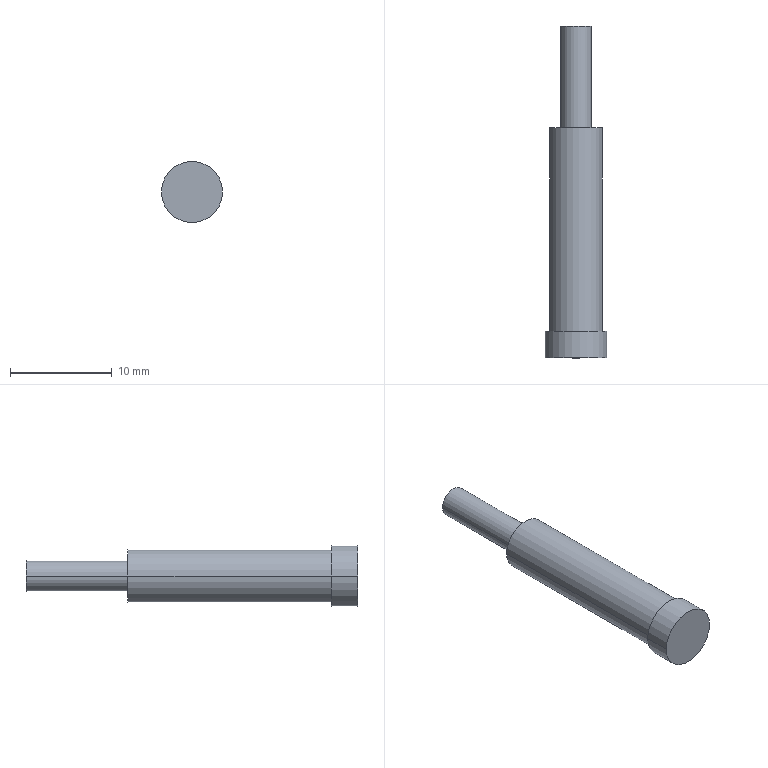Component | SolidWorks | FQ-10-1 | 1 solid | 10 faces | box 6 x 32.6 x 6 mm | volume 569 mm3 | cylinder 6 | plane 4 | commonest cylinder face diameters 3 x2 5.2 x2 6 x2
build123d program:
from build123d import *

# Parameters (mm, degrees)
SKETCH1_R           = 3
BOSS_EXTRUDE1_DEPTH = 2.6
SKETCH2_R           = 2.6
BOSS_EXTRUDE2_DEPTH = 20
SKETCH3_R           = 1.5
BOSS_EXTRUDE3_DEPTH = 10


with BuildPart() as part:
    # Sketch1 → Boss-Extrude1 (new body)
    with BuildSketch(Plane.XY):
        Circle(SKETCH1_R)
    extrude(amount=BOSS_EXTRUDE1_DEPTH)

    # Sketch2 → Boss-Extrude2 (add)
    with BuildSketch(Plane.XY.offset(2.6)):
        Circle(SKETCH2_R)
    extrude(amount=BOSS_EXTRUDE2_DEPTH)

    # Sketch3 → Boss-Extrude3 (add)
    with BuildSketch(Plane.XY.offset(22.6)):
        Circle(SKETCH3_R)
    extrude(amount=BOSS_EXTRUDE3_DEPTH)


solid = part.part

# Placed as in the assembly
solid = solid.moved(Location((-102.663, 0.3959, 98.5), (-90, 0, 0)))
STEP:
#1=COLOUR_RGB('',0.7922,0.8196,0.9333);
#2=FILL_AREA_STYLE_COLOUR('',#1);
#3=FILL_AREA_STYLE('',(#2));
#4=SURFACE_STYLE_FILL_AREA(#3);
#5=SURFACE_SIDE_STYLE('',(#4));
#6=SURFACE_STYLE_USAGE(.BOTH.,#5);
#7=PRESENTATION_STYLE_ASSIGNMENT((#6));
#8=CARTESIAN_POINT('',(-3.983,1.299,3.878));
#9=VERTEX_POINT('',#8);
#10=CARTESIAN_POINT('',(-4.101,1.299,3.878));
#11=VERTEX_POINT('',#10);
#12=CARTESIAN_POINT('',(-4.042,1.299,3.878));
#13=DIRECTION('',(0.,1.,0.));
#14=DIRECTION('',(1.,0.,0.));
#15=AXIS2_PLACEMENT_3D('',#12,#13,#14);
#16=CIRCLE('',#15,0.05906);
#17=EDGE_CURVE('',#9,#11,#16,.T.);
#18=ORIENTED_EDGE('',*,*,#17,.F.);
#19=CARTESIAN_POINT('',(-3.983,0.9054,3.878));
#20=VERTEX_POINT('',#19);
#21=CARTESIAN_POINT('',(-3.983,1.299,3.878));
#22=DIRECTION('',(0.,-1.,0.));
#23=VECTOR('',#22,39.37);
#24=LINE('',#21,#23);
#25=EDGE_CURVE('',#9,#20,#24,.T.);
#26=ORIENTED_EDGE('',*,*,#25,.T.);
#27=CARTESIAN_POINT('',(-4.101,0.9054,3.878));
#28=VERTEX_POINT('',#27);
#29=CARTESIAN_POINT('',(-4.042,0.9054,3.878));
#30=DIRECTION('',(0.,1.,0.));
#31=DIRECTION('',(1.,0.,0.));
#32=AXIS2_PLACEMENT_3D('',#29,#30,#31);
#33=CIRCLE('',#32,0.05906);
#34=EDGE_CURVE('',#20,#28,#33,.T.);
#35=ORIENTED_EDGE('',*,*,#34,.T.);
#36=CARTESIAN_POINT('',(-4.101,1.299,3.878));
#37=DIRECTION('',(0.,-1.,0.));
#38=VECTOR('',#37,39.37);
#39=LINE('',#36,#38);
#40=EDGE_CURVE('',#11,#28,#39,.T.);
#41=ORIENTED_EDGE('',*,*,#40,.F.);
#42=EDGE_LOOP('',(#18,#26,#35,#41));
#43=FACE_OUTER_BOUND('',#42,.T.);
#44=CARTESIAN_POINT('',(-4.042,1.299,3.878));
#45=DIRECTION('',(0.,-1.,0.));
#46=DIRECTION('',(-1.,0.,0.));
#47=AXIS2_PLACEMENT_3D('',#44,#45,#46);
#48=CYLINDRICAL_SURFACE('',#47,0.05906);
#49=ADVANCED_FACE('',(#43),#48,.T.);
#50=CARTESIAN_POINT('',(-3.94,0.9054,3.878));
#51=VERTEX_POINT('',#50);
#52=CARTESIAN_POINT('',(-4.144,0.9054,3.878));
#53=VERTEX_POINT('',#52);
#54=CARTESIAN_POINT('',(-4.042,0.9054,3.878));
#55=DIRECTION('',(0.,1.,0.));
#56=DIRECTION('',(1.,0.,0.));
#57=AXIS2_PLACEMENT_3D('',#54,#55,#56);
#58=CIRCLE('',#57,0.1024);
#59=EDGE_CURVE('',#51,#53,#58,.T.);
#60=ORIENTED_EDGE('',*,*,#59,.F.);
#61=CARTESIAN_POINT('',(-3.94,0.118,3.878));
#62=VERTEX_POINT('',#61);
#63=CARTESIAN_POINT('',(-3.94,0.9054,3.878));
#64=DIRECTION('',(0.,-1.,0.));
#65=VECTOR('',#64,39.37);
#66=LINE('',#63,#65);
#67=EDGE_CURVE('',#51,#62,#66,.T.);
#68=ORIENTED_EDGE('',*,*,#67,.T.);
#69=CARTESIAN_POINT('',(-4.144,0.118,3.878));
#70=VERTEX_POINT('',#69);
#71=CARTESIAN_POINT('',(-4.042,0.118,3.878));
#72=DIRECTION('',(0.,1.,0.));
#73=DIRECTION('',(1.,0.,0.));
#74=AXIS2_PLACEMENT_3D('',#71,#72,#73);
#75=CIRCLE('',#74,0.1024);
#76=EDGE_CURVE('',#62,#70,#75,.T.);
#77=ORIENTED_EDGE('',*,*,#76,.T.);
#78=CARTESIAN_POINT('',(-4.144,0.9054,3.878));
#79=DIRECTION('',(0.,-1.,0.));
#80=VECTOR('',#79,39.37);
#81=LINE('',#78,#80);
#82=EDGE_CURVE('',#53,#70,#81,.T.);
#83=ORIENTED_EDGE('',*,*,#82,.F.);
#84=EDGE_LOOP('',(#60,#68,#77,#83));
#85=FACE_OUTER_BOUND('',#84,.T.);
#86=CARTESIAN_POINT('',(-4.042,0.9054,3.878));
#87=DIRECTION('',(0.,-1.,0.));
#88=DIRECTION('',(-1.,0.,0.));
#89=AXIS2_PLACEMENT_3D('',#86,#87,#88);
#90=CYLINDRICAL_SURFACE('',#89,0.1024);
#91=ADVANCED_FACE('',(#85),#90,.T.);
#92=CARTESIAN_POINT('',(-3.924,0.118,3.878));
#93=VERTEX_POINT('',#92);
#94=CARTESIAN_POINT('',(-4.16,0.118,3.878));
#95=VERTEX_POINT('',#94);
#96=CARTESIAN_POINT('',(-4.042,0.118,3.878));
#97=DIRECTION('',(0.,1.,0.));
#98=DIRECTION('',(1.,0.,0.));
#99=AXIS2_PLACEMENT_3D('',#96,#97,#98);
#100=CIRCLE('',#99,0.1181);
#101=EDGE_CURVE('',#93,#95,#100,.T.);
#102=ORIENTED_EDGE('',*,*,#101,.F.);
#103=CARTESIAN_POINT('',(-3.924,0.01559,3.878));
#104=VERTEX_POINT('',#103);
#105=CARTESIAN_POINT('',(-3.924,0.118,3.878));
#106=DIRECTION('',(0.,-1.,0.));
#107=VECTOR('',#106,39.37);
#108=LINE('',#105,#107);
#109=EDGE_CURVE('',#93,#104,#108,.T.);
#110=ORIENTED_EDGE('',*,*,#109,.T.);
#111=CARTESIAN_POINT('',(-4.16,0.01559,3.878));
#112=VERTEX_POINT('',#111);
#113=CARTESIAN_POINT('',(-4.042,0.01559,3.878));
#114=DIRECTION('',(0.,1.,0.));
#115=DIRECTION('',(1.,0.,0.));
#116=AXIS2_PLACEMENT_3D('',#113,#114,#115);
#117=CIRCLE('',#116,0.1181);
#118=EDGE_CURVE('',#104,#112,#117,.T.);
#119=ORIENTED_EDGE('',*,*,#118,.T.);
#120=CARTESIAN_POINT('',(-4.16,0.118,3.878));
#121=DIRECTION('',(0.,-1.,0.));
#122=VECTOR('',#121,39.37);
#123=LINE('',#120,#122);
#124=EDGE_CURVE('',#95,#112,#123,.T.);
#125=ORIENTED_EDGE('',*,*,#124,.F.);
#126=EDGE_LOOP('',(#102,#110,#119,#125));
#127=FACE_OUTER_BOUND('',#126,.T.);
#128=CARTESIAN_POINT('',(-4.042,0.118,3.878));
#129=DIRECTION('',(0.,-1.,0.));
#130=DIRECTION('',(-1.,0.,0.));
#131=AXIS2_PLACEMENT_3D('',#128,#129,#130);
#132=CYLINDRICAL_SURFACE('',#131,0.1181);
#133=ADVANCED_FACE('',(#127),#132,.T.);
#134=ORIENTED_EDGE('',*,*,#109,.F.);
#135=CARTESIAN_POINT('',(-4.042,0.118,3.878));
#136=DIRECTION('',(0.,1.,0.));
#137=DIRECTION('',(1.,0.,0.));
#138=AXIS2_PLACEMENT_3D('',#135,#136,#137);
#139=CIRCLE('',#138,0.1181);
#140=EDGE_CURVE('',#95,#93,#139,.T.);
#141=ORIENTED_EDGE('',*,*,#140,.F.);
#142=ORIENTED_EDGE('',*,*,#124,.T.);
#143=CARTESIAN_POINT('',(-4.042,0.01559,3.878));
#144=DIRECTION('',(0.,1.,0.));
#145=DIRECTION('',(1.,0.,0.));
#146=AXIS2_PLACEMENT_3D('',#143,#144,#145);
#147=CIRCLE('',#146,0.1181);
#148=EDGE_CURVE('',#112,#104,#147,.T.);
#149=ORIENTED_EDGE('',*,*,#148,.T.);
#150=EDGE_LOOP('',(#134,#141,#142,#149));
#151=FACE_OUTER_BOUND('',#150,.T.);
#152=CARTESIAN_POINT('',(-4.042,0.118,3.878));
#153=DIRECTION('',(0.,-1.,0.));
#154=DIRECTION('',(-1.,0.,0.));
#155=AXIS2_PLACEMENT_3D('',#152,#153,#154);
#156=CYLINDRICAL_SURFACE('',#155,0.1181);
#157=ADVANCED_FACE('',(#151),#156,.T.);
#158=CARTESIAN_POINT('',(-4.042,0.118,3.878));
#159=DIRECTION('',(0.,1.,0.));
#160=DIRECTION('',(1.,0.,0.));
#161=AXIS2_PLACEMENT_3D('',#158,#159,#160);
#162=CIRCLE('',#161,0.1024);
#163=EDGE_CURVE('',#70,#62,#162,.T.);
#164=ORIENTED_EDGE('',*,*,#163,.F.);
#165=ORIENTED_EDGE('',*,*,#76,.F.);
#166=EDGE_LOOP('',(#164,#165));
#167=FACE_BOUND('',#166,.T.);
#168=ORIENTED_EDGE('',*,*,#140,.T.);
#169=ORIENTED_EDGE('',*,*,#101,.T.);
#170=EDGE_LOOP('',(#168,#169));
#171=FACE_OUTER_BOUND('',#170,.T.);
#172=CARTESIAN_POINT('',(-4.042,0.118,3.878));
#173=DIRECTION('',(0.,1.,0.));
#174=DIRECTION('',(1.,0.,0.));
#175=AXIS2_PLACEMENT_3D('',#172,#173,#174);
#176=PLANE('',#175);
#177=ADVANCED_FACE('',(#167,#171),#176,.T.);
#178=ORIENTED_EDGE('',*,*,#148,.F.);
#179=ORIENTED_EDGE('',*,*,#118,.F.);
#180=EDGE_LOOP('',(#178,#179));
#181=FACE_OUTER_BOUND('',#180,.T.);
#182=CARTESIAN_POINT('',(-4.042,0.01559,3.878));
#183=DIRECTION('',(0.,1.,0.));
#184=DIRECTION('',(1.,0.,0.));
#185=AXIS2_PLACEMENT_3D('',#182,#183,#184);
#186=PLANE('',#185);
#187=ADVANCED_FACE('',(#181),#186,.F.);
#188=ORIENTED_EDGE('',*,*,#67,.F.);
#189=CARTESIAN_POINT('',(-4.042,0.9054,3.878));
#190=DIRECTION('',(0.,1.,0.));
#191=DIRECTION('',(1.,0.,0.));
#192=AXIS2_PLACEMENT_3D('',#189,#190,#191);
#193=CIRCLE('',#192,0.1024);
#194=EDGE_CURVE('',#53,#51,#193,.T.);
#195=ORIENTED_EDGE('',*,*,#194,.F.);
#196=ORIENTED_EDGE('',*,*,#82,.T.);
#197=ORIENTED_EDGE('',*,*,#163,.T.);
#198=EDGE_LOOP('',(#188,#195,#196,#197));
#199=FACE_OUTER_BOUND('',#198,.T.);
#200=CARTESIAN_POINT('',(-4.042,0.9054,3.878));
#201=DIRECTION('',(0.,-1.,0.));
#202=DIRECTION('',(-1.,0.,0.));
#203=AXIS2_PLACEMENT_3D('',#200,#201,#202);
#204=CYLINDRICAL_SURFACE('',#203,0.1024);
#205=ADVANCED_FACE('',(#199),#204,.T.);
#206=CARTESIAN_POINT('',(-4.042,0.9054,3.878));
#207=DIRECTION('',(0.,1.,0.));
#208=DIRECTION('',(1.,0.,0.));
#209=AXIS2_PLACEMENT_3D('',#206,#207,#208);
#210=CIRCLE('',#209,0.05906);
#211=EDGE_CURVE('',#28,#20,#210,.T.);
#212=ORIENTED_EDGE('',*,*,#211,.F.);
#213=ORIENTED_EDGE('',*,*,#34,.F.);
#214=EDGE_LOOP('',(#212,#213));
#215=FACE_BOUND('',#214,.T.);
#216=ORIENTED_EDGE('',*,*,#194,.T.);
#217=ORIENTED_EDGE('',*,*,#59,.T.);
#218=EDGE_LOOP('',(#216,#217));
#219=FACE_OUTER_BOUND('',#218,.T.);
#220=CARTESIAN_POINT('',(-4.042,0.9054,3.878));
#221=DIRECTION('',(0.,1.,0.));
#222=DIRECTION('',(1.,0.,0.));
#223=AXIS2_PLACEMENT_3D('',#220,#221,#222);
#224=PLANE('',#223);
#225=ADVANCED_FACE('',(#215,#219),#224,.T.);
#226=ORIENTED_EDGE('',*,*,#25,.F.);
#227=CARTESIAN_POINT('',(-4.042,1.299,3.878));
#228=DIRECTION('',(0.,1.,0.));
#229=DIRECTION('',(1.,0.,0.));
#230=AXIS2_PLACEMENT_3D('',#227,#228,#229);
#231=CIRCLE('',#230,0.05906);
#232=EDGE_CURVE('',#11,#9,#231,.T.);
#233=ORIENTED_EDGE('',*,*,#232,.F.);
#234=ORIENTED_EDGE('',*,*,#40,.T.);
#235=ORIENTED_EDGE('',*,*,#211,.T.);
#236=EDGE_LOOP('',(#226,#233,#234,#235));
#237=FACE_OUTER_BOUND('',#236,.T.);
#238=CARTESIAN_POINT('',(-4.042,1.299,3.878));
#239=DIRECTION('',(0.,-1.,0.));
#240=DIRECTION('',(-1.,0.,0.));
#241=AXIS2_PLACEMENT_3D('',#238,#239,#240);
#242=CYLINDRICAL_SURFACE('',#241,0.05906);
#243=ADVANCED_FACE('',(#237),#242,.T.);
#244=ORIENTED_EDGE('',*,*,#232,.T.);
#245=ORIENTED_EDGE('',*,*,#17,.T.);
#246=EDGE_LOOP('',(#244,#245));
#247=FACE_OUTER_BOUND('',#246,.T.);
#248=CARTESIAN_POINT('',(-4.042,1.299,3.878));
#249=DIRECTION('',(0.,1.,0.));
#250=DIRECTION('',(1.,0.,0.));
#251=AXIS2_PLACEMENT_3D('',#248,#249,#250);
#252=PLANE('',#251);
#253=ADVANCED_FACE('',(#247),#252,.T.);
#254=CLOSED_SHELL('',(#49,#91,#133,#157,#177,#187,#205,#225,#243,#253));
#255=MANIFOLD_SOLID_BREP('',#254);
#256=STYLED_ITEM('',(#7),#255);
#257=PRESENTATION_LAYER_ASSIGNMENT('','',(#256));
#258=(LENGTH_UNIT()NAMED_UNIT(*)SI_UNIT($,.METRE.));
#259=LENGTH_MEASURE_WITH_UNIT(LENGTH_MEASURE(0.0254),#258);
#260=DIMENSIONAL_EXPONENTS(1.,0.,0.,0.,0.,0.,0.);
#261=(CONVERSION_BASED_UNIT('',#259)LENGTH_UNIT()NAMED_UNIT(#260));
#262=UNCERTAINTY_MEASURE_WITH_UNIT(LENGTH_MEASURE(0.00001),#261,'','');
#263=(NAMED_UNIT(*)PLANE_ANGLE_UNIT()SI_UNIT($,.RADIAN.));
#264=(NAMED_UNIT(*)SI_UNIT($,.STERADIAN.)SOLID_ANGLE_UNIT());
#265=(GEOMETRIC_REPRESENTATION_CONTEXT(3)GLOBAL_UNCERTAINTY_ASSIGNED_CONTEXT((#262))GLOBAL_UNIT_ASSIGNED_CONTEXT((#261,#263,#264))REPRESENTATION_CONTEXT('',''));
#266=MECHANICAL_DESIGN_GEOMETRIC_PRESENTATION_REPRESENTATION('',(#256),#265);
#267=CARTESIAN_POINT('',(0.,0.,0.));
#268=DIRECTION('',(0.,0.,1.));
#269=DIRECTION('',(1.,0.,0.));
#270=AXIS2_PLACEMENT_3D('',#267,#268,#269);
#271=(LENGTH_UNIT()NAMED_UNIT(*)SI_UNIT($,.METRE.));
#272=LENGTH_MEASURE_WITH_UNIT(LENGTH_MEASURE(0.0254),#271);
#273=DIMENSIONAL_EXPONENTS(1.,0.,0.,0.,0.,0.,0.);
#274=(CONVERSION_BASED_UNIT('',#272)LENGTH_UNIT()NAMED_UNIT(#273));
#275=UNCERTAINTY_MEASURE_WITH_UNIT(LENGTH_MEASURE(0.00001),#274,'','');
#276=(NAMED_UNIT(*)PLANE_ANGLE_UNIT()SI_UNIT($,.RADIAN.));
#277=(NAMED_UNIT(*)SI_UNIT($,.STERADIAN.)SOLID_ANGLE_UNIT());
#278=(GEOMETRIC_REPRESENTATION_CONTEXT(3)GLOBAL_UNCERTAINTY_ASSIGNED_CONTEXT((#275))GLOBAL_UNIT_ASSIGNED_CONTEXT((#274,#276,#277))REPRESENTATION_CONTEXT('',''));
#279=ADVANCED_BREP_SHAPE_REPRESENTATION('',(#255,#270),#278);